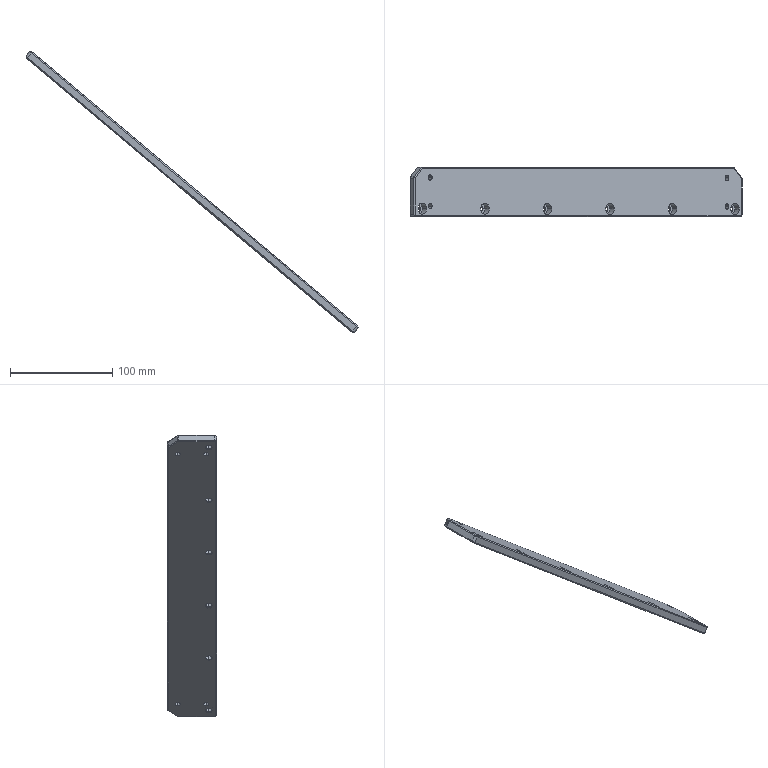Component | SolidWorks | 04ReinforcingRib-1 | 1 solid | 76 faces | box 325.16 x 48 x 275.34 mm | volume 154791 mm3 | cylinder 38 | plane 26 | cone 12 | commonest cylinder face diameters 11 x12 6.6 x12 5 x8 4 x6 | material Aviation Aluminum-7075
build123d program:
from build123d import *

# Parameters (mm, degrees)
SKETCH1_W                                          = 420
SKETCH1_H                                          = 48
BOSS_EXTRUDE1_DEPTH                                = 8
CUT_EXTRUDE1_REACH                                 = 424.81
HOLE_SIZE_ACCORDING_TO_TYPE_1_OF_HEXAG_D           = 6.6
HOLE_SIZE_ACCORDING_TO_TYPE_1_OF_HEXAG_CBORE_D     = 11
HOLE_SIZE_ACCORDING_TO_TYPE_1_OF_HEXAG_CBORE_DEPTH = 6.8
FILLET1_R                                          = 2
M6_TAPPED_HOLE1_AT_2_COUNT                         = 2
M6_TAPPED_HOLE1_AT_2_PITCH                         = 28
CHAMFER1_SIZE                                      = 1


with BuildPart() as part:
    # Sketch1 → Boss-Extrude1 (new body)
    with BuildSketch(Plane.XY):
        with Locations((210, -24)):
            Rectangle(SKETCH1_W, SKETCH1_H)
    extrude(amount=BOSS_EXTRUDE1_DEPTH)

    # Sketch3 → Cut-Extrude1 (cut, up to next)
    with BuildSketch(Plane.XY.offset(8), mode=Mode.PRIVATE) as cut_extrude1_sk1:
        Polygon((0, -38), (10, -48), (0, -48), align=None)
    cut_extrude1_tool1 = extrude(cut_extrude1_sk1.sketch, amount=-CUT_EXTRUDE1_REACH, mode=Mode.PRIVATE) & part.part
    # Sketch3 → Cut-Extrude1 (cut, up to next)
    with BuildSketch(Plane.XY.offset(8), mode=Mode.PRIVATE) as cut_extrude1_sk2:
        Polygon((420, -38), (410, -48), (420, -48), align=None)
    cut_extrude1_tool2 = extrude(cut_extrude1_sk2.sketch, amount=-CUT_EXTRUDE1_REACH, mode=Mode.PRIVATE) & part.part
    add(cut_extrude1_tool1.solids().sort_by_distance((3.333, -44.667, 8))[0], mode=Mode.SUBTRACT)
    add(cut_extrude1_tool2.solids().sort_by_distance((416.667, -44.667, 8))[0], mode=Mode.SUBTRACT)

    # Hole Size _According to_ Type 1 of Hexag (through all)
    with Locations(Plane(origin=(10, -7.5, 8), x_dir=(1, 0, 0), z_dir=(0, 0, 1))):
        with Locations((0, 0), (160, 0), (240, 0), (400, 0), (80, 0), (320, 0)):
            CounterBoreHole(HOLE_SIZE_ACCORDING_TO_TYPE_1_OF_HEXAG_D / 2, HOLE_SIZE_ACCORDING_TO_TYPE_1_OF_HEXAG_CBORE_D / 2, HOLE_SIZE_ACCORDING_TO_TYPE_1_OF_HEXAG_CBORE_DEPTH)

    # Fillet1
    fillet1_edges = [part.edges().sort_by_distance(p)[0] for p in [
        (0, -38, 4),
        (10, -48, 4),
        (420, -38, 4),
        (410, -48, 4),
        (0, 0, 4),
        (420, 0, 4),
    ]]
    fillet(fillet1_edges, radius=FILLET1_R)

    # Sketch5 → M6 Tapped Hole1 (revolve, cut)
    with BuildSketch(Plane(origin=(400, -38, 8), x_dir=(0, -1, 0), z_dir=(1, 0, 0))):
        Polygon((0, 0), (0, 16.502), (2.5, 15), (2.5, 0), align=None)
    m6_tapped_hole1 = revolve(axis=Axis((400, -38, 14.35), (0, 0, -1)), mode=Mode.SUBTRACT)

    # M6 Tapped Hole1 at 2: M6 Tapped Hole1 ×2
    with Locations(*[(0, i * M6_TAPPED_HOLE1_AT_2_PITCH, 0) for i in range(1, M6_TAPPED_HOLE1_AT_2_COUNT)]):
        add(m6_tapped_hole1, mode=Mode.SUBTRACT)

    # Mirror2: M6 Tapped Hole1 across plane
    add(m6_tapped_hole1.mirror(Plane.ZY.offset(-210)), mode=Mode.SUBTRACT)

    # Mirror2 copy 1 sketch → Mirror2 copy 1 (revolve, cut)
    with BuildSketch(Plane(origin=(20, -10, 8), x_dir=(0, -1, 0), z_dir=(-1, 0, 0))):
        Polygon((0, 0), (0, -16.502), (2.5, -15), (2.5, 0), align=None)
    revolve(axis=Axis((20, -10, 14.35), (0, 0, 1)), mode=Mode.SUBTRACT)

    # Chamfer1
    chamfer1_edges = [part.edges().sort_by_distance(p)[0] for p in [
        (210, 0, 0),
        (0.1522, -37.937, 0),
        (10.063, -47.848, 0),
        (0.5858, -0.5858, 0),
        (419.414, -0.5858, 0),
        (409.937, -47.848, 0),
        (419.848, -37.937, 0),
        (415, -43, 0),
        (415, -43, 8),
        (5, -43, 8),
        (210, -48, 8),
        (420, -19.586, 8),
        (210, 0, 8),
        (0, -19.586, 8),
        (0.1522, -37.937, 8),
        (10.063, -47.848, 8),
        (0.5858, -0.5858, 8),
        (419.414, -0.5858, 8),
        (409.937, -47.848, 8),
        (419.848, -37.937, 8),
        (420, -19.586, 0),
        (210, -48, 0),
        (5, -43, 0),
        (0, -19.586, 0),
    ]]
    chamfer(chamfer1_edges, length=CHAMFER1_SIZE)


solid = part.part

# Placed as in the assembly
solid = solid.moved(Location((2.462, 149.645, -322.469), (0, 40.095, 180)))